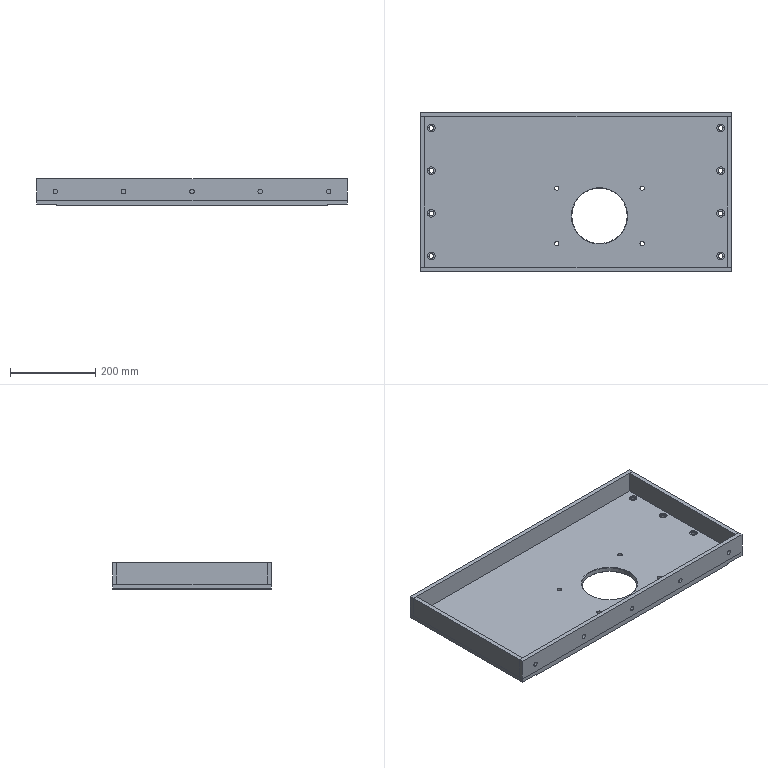Component | SolidWorks | MovingVerticalPlate3-1 | 5 solids | 113 faces | volume 4065064 mm3 | cylinder 62 | plane 47 | cone 4 | commonest cylinder face diameters 18 x26 11 x26 10.2 x8 130 x2